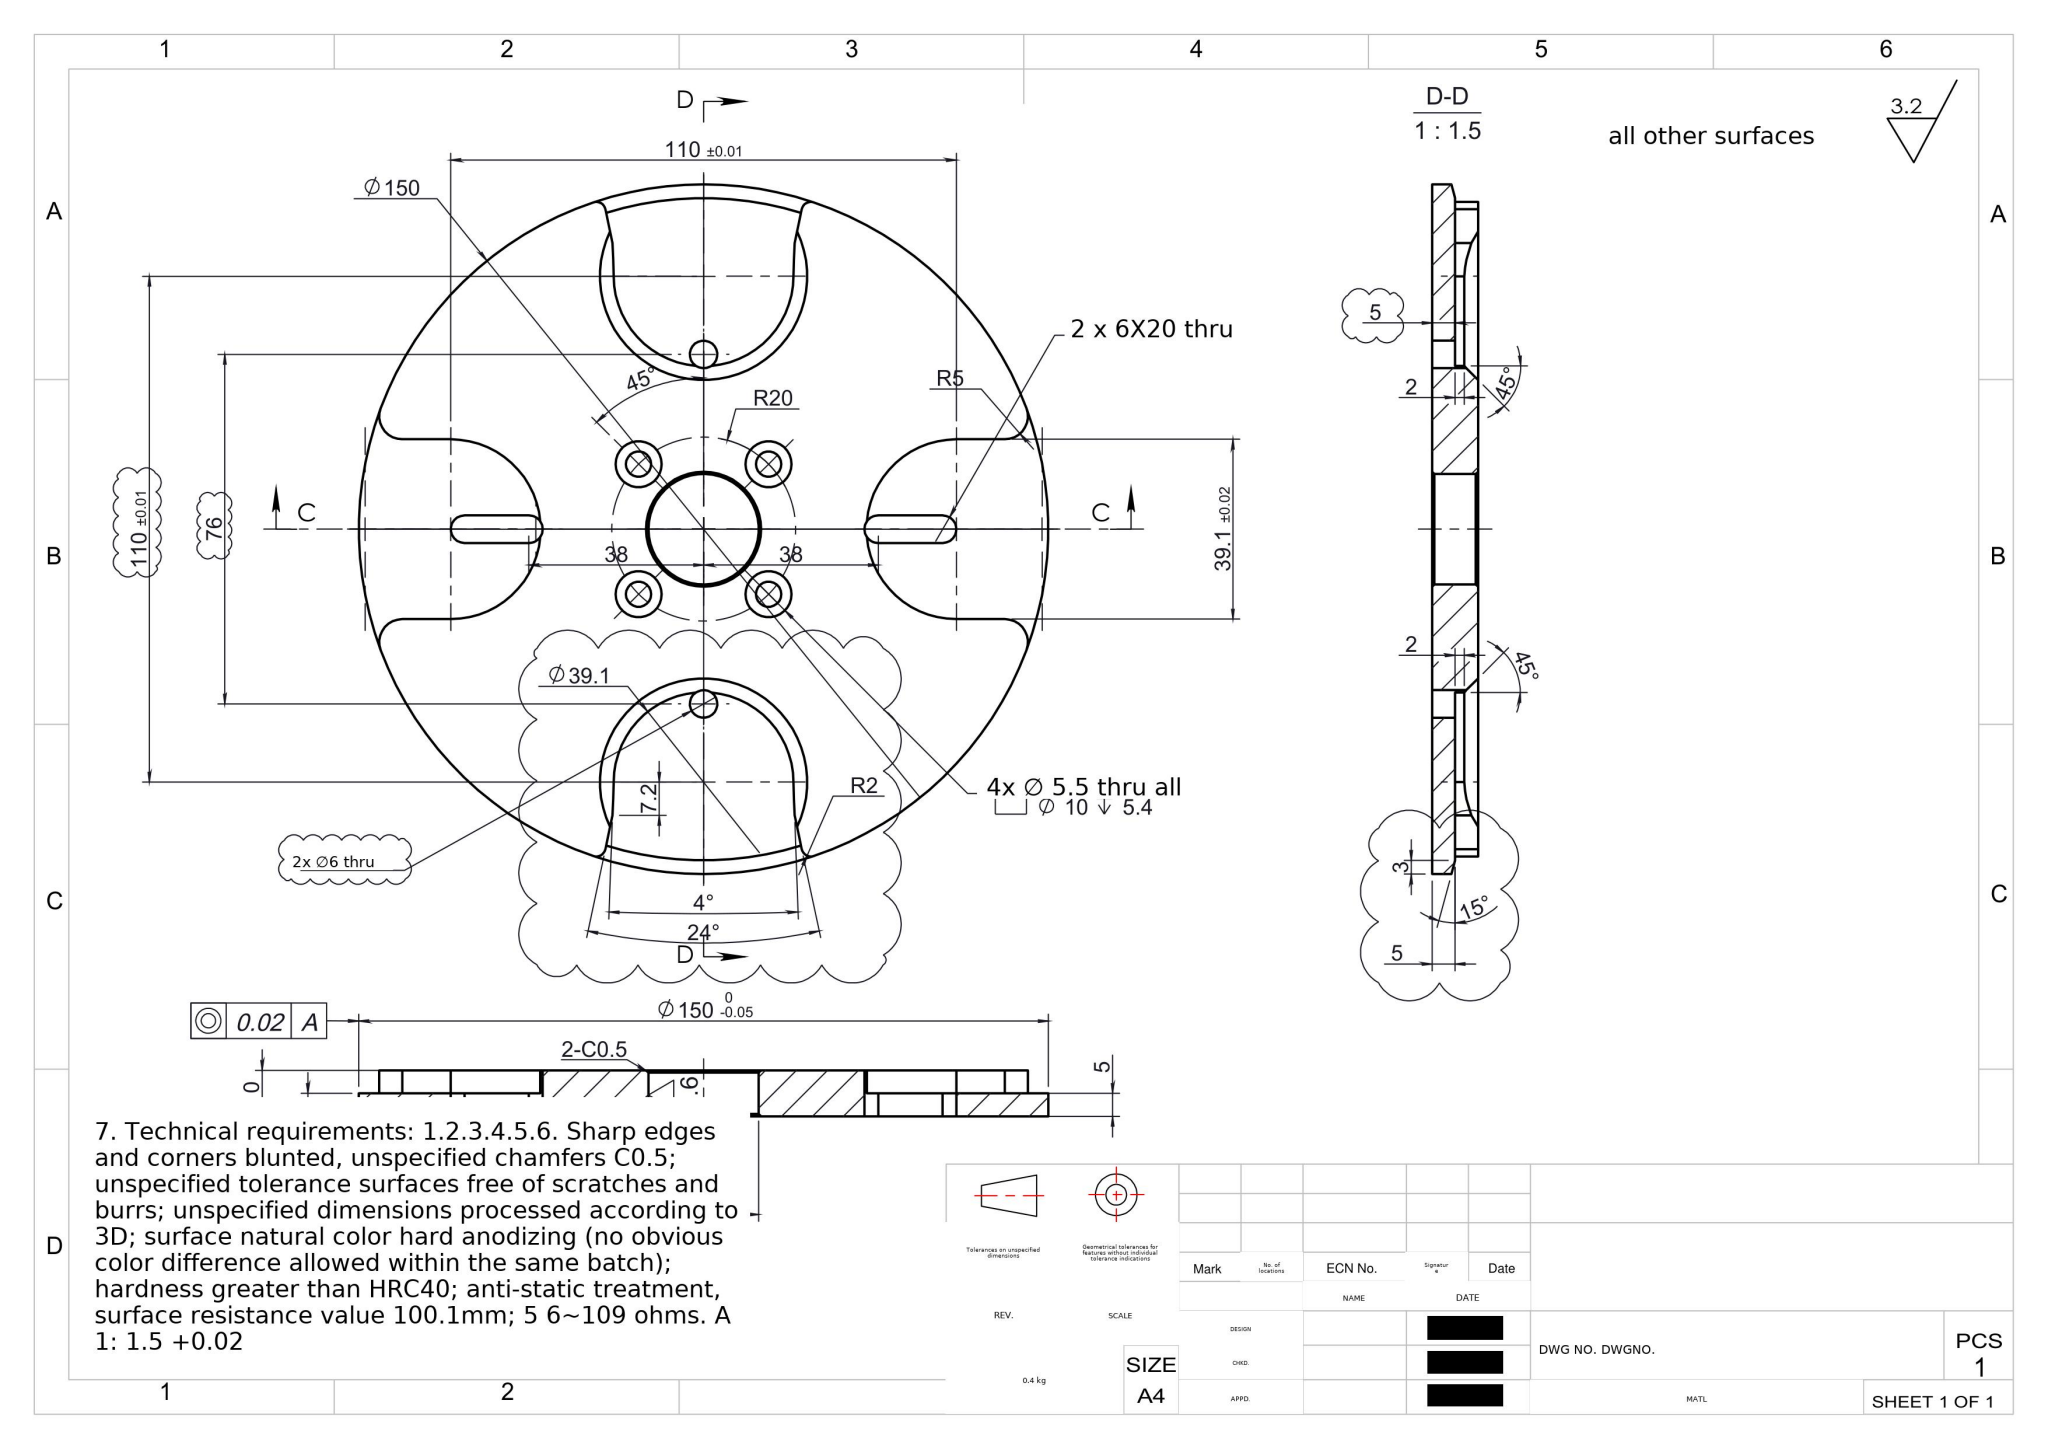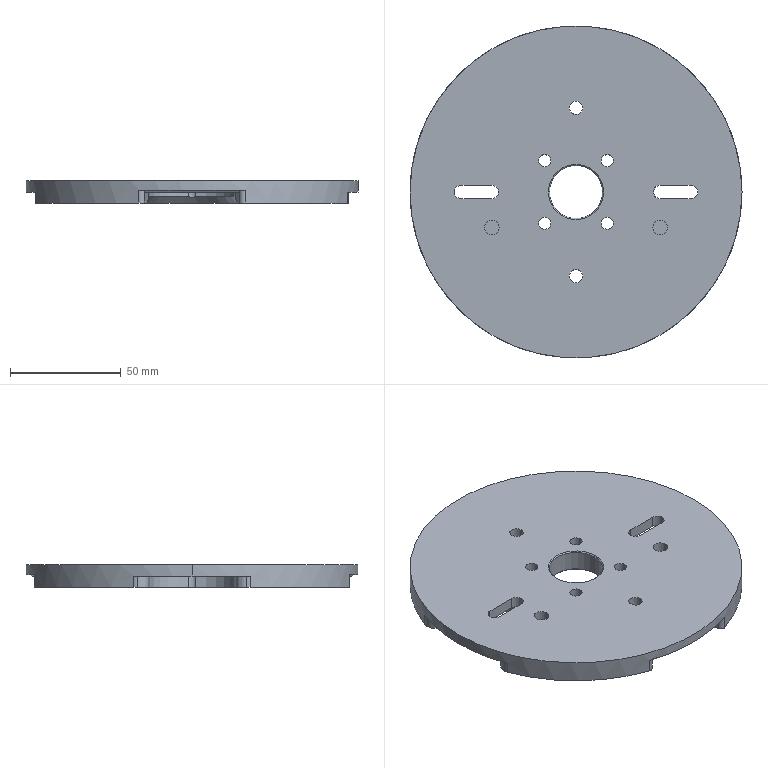Part | SolidWorks | mm | 1 solid | 92 faces | box 150 x 150 x 10 mm | volume 139997 mm3 | cylinder 52 | plane 28 | cone 12 | commonest cylinder face diameters 10 x14 6 x10 5.5 x8 39.1 x8 6.6 x4 4 x4 24 x2 150 x2